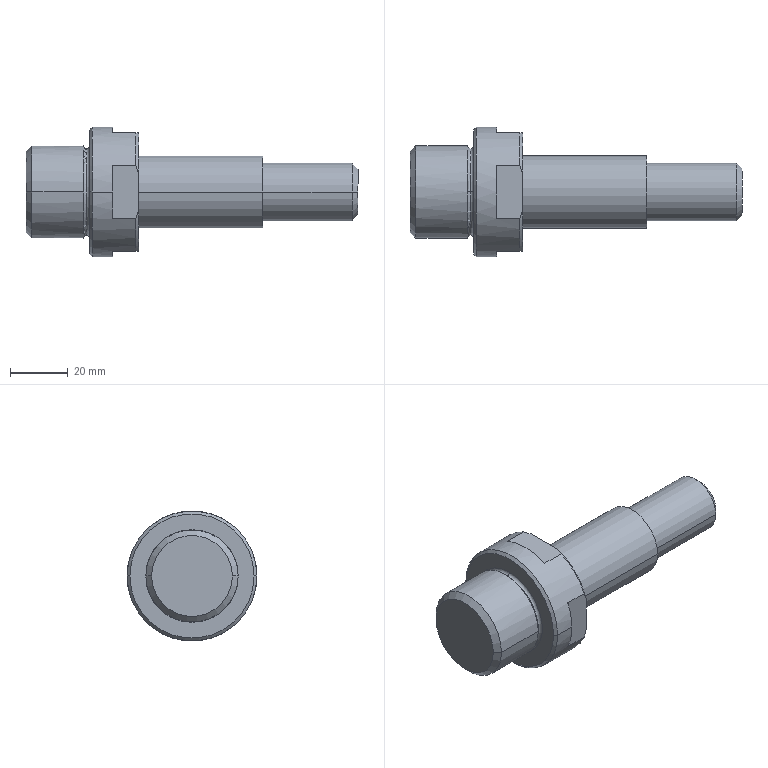Component | SolidWorks | FE5-226--a_b-1 | 1 solid | 35 faces | box 115 x 45 x 45 mm | volume 74739 mm3 | plane 13 | cone 10 | cylinder 8 | torus 4 | commonest cylinder face diameters 32 x2 20 x2 25 x2 45 x2
build123d program:
from build123d import *

# Parameters (mm, degrees)
SKETCH2_R       = 1
CHAMFER2_1_SIZE = 2
CHAMFER1_1_SIZE = 1
SKETCH3_W       = 30
SKETCH3_H       = 5
SKETCH3_W_2     = 5
SKETCH3_H_2     = 30
EXTRUDE1_DEPTH  = 9


with BuildPart() as part:
    # Sketch1 → Revolve1 (revolve)
    with BuildSketch(Plane(origin=(0, 0, 0), x_dir=(0, 0, -1), z_dir=(1, 0, 0))):
        Polygon((-115, 0), (-115, 16), (-93, 16), (-93, 22.5), (-76, 22.5), (-76, 12.5), (-33, 12.5), (-33, 10), (0, 10), (0, 0), align=None)
    revolve(axis=Axis((0, 0, 0), (0, 0, 1)))

    # Sketch2 → Cut-Revolve1 (revolve, cut)
    with BuildSketch(Plane(origin=(0, 0, 0), x_dir=(0, 0, -1), z_dir=(1, 0, 0)), mode=Mode.PRIVATE) as cut_revolve1_sk:
        with Locations((-94, 16)):
            Circle(SKETCH2_R)
    revolve(cut_revolve1_sk.sketch.rotate(Axis((0, 0, 0), (0, 0, 1)), 90), axis=Axis((0, 0, 0), (0, 0, 1)), mode=Mode.SUBTRACT)

    # Chamfer2-1
    chamfer2_1_edges = [part.edges().sort_by_distance(p)[0] for p in [
        (0, -16, 115),
        (0, -10, 0),
    ]]
    chamfer(chamfer2_1_edges, length=CHAMFER2_1_SIZE)

    # Chamfer1-1
    chamfer1_1_edges = [part.edges().sort_by_distance(p)[0] for p in [
        (0, -22.5, 76),
        (0, -22.5, 93),
    ]]
    chamfer(chamfer1_1_edges, length=CHAMFER1_1_SIZE)

    # Sketch3 → Extrude1 (cut)
    with BuildSketch(Plane(origin=(0, 0, 76), x_dir=(-1, 0, 0), z_dir=(0, 0, -1))):
        with Locations((0, 23)):
            Rectangle(SKETCH3_W, SKETCH3_H)
        with Locations((23, 0)):
            Rectangle(SKETCH3_W_2, SKETCH3_H_2)
        with Locations((-23, 0)):
            Rectangle(SKETCH3_W_2, SKETCH3_H_2)
        with Locations((0, -23)):
            Rectangle(SKETCH3_W, SKETCH3_H)
    extrude(amount=-EXTRUDE1_DEPTH, mode=Mode.SUBTRACT)


solid = part.part

# Placed as in the assembly
solid = solid.moved(Location((100, 81, -460), (0, -90, 0)))
STEP:
#1=CARTESIAN_POINT('',(0.2756,3.189,-18.74));
#2=VERTEX_POINT('',#1);
#3=CARTESIAN_POINT('',(0.2362,3.189,-18.701));
#4=VERTEX_POINT('',#3);
#5=CARTESIAN_POINT('',(0.2362,3.189,-18.74));
#6=DIRECTION('',(-0.,-1.,-0.));
#7=DIRECTION('',(1.,0.,0.));
#8=AXIS2_PLACEMENT_3D('',#5,#6,#7);
#9=CIRCLE('',#8,0.03937);
#10=EDGE_CURVE('',#2,#4,#9,.T.);
#11=ORIENTED_EDGE('',*,*,#10,.T.);
#12=CARTESIAN_POINT('',(0.2362,3.189,-17.52));
#13=VERTEX_POINT('',#12);
#14=CARTESIAN_POINT('',(0.2362,3.189,-18.11));
#15=DIRECTION('',(1.,-0.,-0.));
#16=DIRECTION('',(-0.,0.,-1.));
#17=AXIS2_PLACEMENT_3D('',#14,#15,#16);
#18=CIRCLE('',#17,0.5906);
#19=EDGE_CURVE('',#4,#13,#18,.T.);
#20=ORIENTED_EDGE('',*,*,#19,.T.);
#21=CARTESIAN_POINT('',(0.2756,3.189,-17.48));
#22=VERTEX_POINT('',#21);
#23=CARTESIAN_POINT('',(0.2362,3.189,-17.48));
#24=DIRECTION('',(0.,1.,-0.));
#25=DIRECTION('',(-1.,0.,0.));
#26=AXIS2_PLACEMENT_3D('',#23,#24,#25);
#27=CIRCLE('',#26,0.03937);
#28=EDGE_CURVE('',#22,#13,#27,.T.);
#29=ORIENTED_EDGE('',*,*,#28,.F.);
#30=CARTESIAN_POINT('',(0.2756,3.189,-18.11));
#31=DIRECTION('',(1.,-0.,-0.));
#32=DIRECTION('',(-0.,0.,-1.));
#33=AXIS2_PLACEMENT_3D('',#30,#31,#32);
#34=CIRCLE('',#33,0.6299);
#35=EDGE_CURVE('',#2,#22,#34,.T.);
#36=ORIENTED_EDGE('',*,*,#35,.F.);
#37=EDGE_LOOP('',(#11,#20,#29,#36));
#38=FACE_OUTER_BOUND('',#37,.T.);
#39=CARTESIAN_POINT('',(0.2362,3.189,-18.11));
#40=DIRECTION('',(1.,-0.,-0.));
#41=DIRECTION('',(-0.,0.,-1.));
#42=AXIS2_PLACEMENT_3D('',#39,#40,#41);
#43=TOROIDAL_SURFACE('',#42,0.6299,0.03937);
#44=ADVANCED_FACE('',(#38),#43,.F.);
#45=ORIENTED_EDGE('',*,*,#28,.T.);
#46=CARTESIAN_POINT('',(0.2362,3.189,-18.11));
#47=DIRECTION('',(1.,-0.,-0.));
#48=DIRECTION('',(-0.,0.,-1.));
#49=AXIS2_PLACEMENT_3D('',#46,#47,#48);
#50=CIRCLE('',#49,0.5906);
#51=EDGE_CURVE('',#13,#4,#50,.T.);
#52=ORIENTED_EDGE('',*,*,#51,.T.);
#53=ORIENTED_EDGE('',*,*,#10,.F.);
#54=CARTESIAN_POINT('',(0.2756,3.189,-18.11));
#55=DIRECTION('',(1.,-0.,-0.));
#56=DIRECTION('',(-0.,0.,-1.));
#57=AXIS2_PLACEMENT_3D('',#54,#55,#56);
#58=CIRCLE('',#57,0.6299);
#59=EDGE_CURVE('',#22,#2,#58,.T.);
#60=ORIENTED_EDGE('',*,*,#59,.F.);
#61=EDGE_LOOP('',(#45,#52,#53,#60));
#62=FACE_OUTER_BOUND('',#61,.T.);
#63=CARTESIAN_POINT('',(0.2362,3.189,-18.11));
#64=DIRECTION('',(1.,-0.,-0.));
#65=DIRECTION('',(-0.,0.,-1.));
#66=AXIS2_PLACEMENT_3D('',#63,#64,#65);
#67=TOROIDAL_SURFACE('',#66,0.6299,0.03937);
#68=ADVANCED_FACE('',(#62),#67,.F.);
#69=CARTESIAN_POINT('',(0.2756,2.343,-18.11));
#70=VERTEX_POINT('',#69);
#71=CARTESIAN_POINT('',(0.2756,4.035,-18.11));
#72=VERTEX_POINT('',#71);
#73=CARTESIAN_POINT('',(0.2756,3.189,-18.11));
#74=DIRECTION('',(-1.,0.,0.));
#75=DIRECTION('',(0.,-1.,0.));
#76=AXIS2_PLACEMENT_3D('',#73,#74,#75);
#77=CIRCLE('',#76,0.8465);
#78=EDGE_CURVE('',#70,#72,#77,.T.);
#79=ORIENTED_EDGE('',*,*,#78,.F.);
#80=CARTESIAN_POINT('',(0.315,2.303,-18.11));
#81=VERTEX_POINT('',#80);
#82=CARTESIAN_POINT('',(0.315,2.303,-18.11));
#83=DIRECTION('',(0.7071,-0.7071,-0.));
#84=VECTOR('',#83,39.37);
#85=LINE('',#82,#84);
#86=EDGE_CURVE('',#70,#81,#85,.T.);
#87=ORIENTED_EDGE('',*,*,#86,.T.);
#88=CARTESIAN_POINT('',(0.315,4.075,-18.11));
#89=VERTEX_POINT('',#88);
#90=CARTESIAN_POINT('',(0.315,3.189,-18.11));
#91=DIRECTION('',(1.,-0.,-0.));
#92=DIRECTION('',(0.,-1.,0.));
#93=AXIS2_PLACEMENT_3D('',#90,#91,#92);
#94=CIRCLE('',#93,0.8858);
#95=EDGE_CURVE('',#89,#81,#94,.T.);
#96=ORIENTED_EDGE('',*,*,#95,.F.);
#97=CARTESIAN_POINT('',(0.315,4.075,-18.11));
#98=DIRECTION('',(0.7071,0.7071,-0.));
#99=VECTOR('',#98,39.37);
#100=LINE('',#97,#99);
#101=EDGE_CURVE('',#72,#89,#100,.T.);
#102=ORIENTED_EDGE('',*,*,#101,.F.);
#103=EDGE_LOOP('',(#79,#87,#96,#102));
#104=FACE_OUTER_BOUND('',#103,.T.);
#105=CARTESIAN_POINT('',(0.315,3.189,-18.11));
#106=DIRECTION('',(1.,-0.,-0.));
#107=DIRECTION('',(0.,1.,0.));
#108=AXIS2_PLACEMENT_3D('',#105,#106,#107);
#109=CONICAL_SURFACE('',#108,0.8858,0.7854);
#110=ADVANCED_FACE('',(#104),#109,.T.);
#111=CARTESIAN_POINT('',(-0.5906,2.638,-18.11));
#112=VERTEX_POINT('',#111);
#113=CARTESIAN_POINT('',(-0.5906,3.74,-18.11));
#114=VERTEX_POINT('',#113);
#115=CARTESIAN_POINT('',(-0.5906,3.189,-18.11));
#116=DIRECTION('',(-1.,0.,0.));
#117=DIRECTION('',(0.,-1.,0.));
#118=AXIS2_PLACEMENT_3D('',#115,#116,#117);
#119=CIRCLE('',#118,0.5512);
#120=EDGE_CURVE('',#112,#114,#119,.T.);
#121=ORIENTED_EDGE('',*,*,#120,.F.);
#122=CARTESIAN_POINT('',(-0.5118,2.559,-18.11));
#123=VERTEX_POINT('',#122);
#124=CARTESIAN_POINT('',(-0.5118,2.559,-18.11));
#125=DIRECTION('',(0.7071,-0.7071,-0.));
#126=VECTOR('',#125,39.37);
#127=LINE('',#124,#126);
#128=EDGE_CURVE('',#112,#123,#127,.T.);
#129=ORIENTED_EDGE('',*,*,#128,.T.);
#130=CARTESIAN_POINT('',(-0.5118,3.819,-18.11));
#131=VERTEX_POINT('',#130);
#132=CARTESIAN_POINT('',(-0.5118,3.189,-18.11));
#133=DIRECTION('',(1.,0.,-0.));
#134=DIRECTION('',(0.,-1.,0.));
#135=AXIS2_PLACEMENT_3D('',#132,#133,#134);
#136=CIRCLE('',#135,0.6299);
#137=EDGE_CURVE('',#131,#123,#136,.T.);
#138=ORIENTED_EDGE('',*,*,#137,.F.);
#139=CARTESIAN_POINT('',(-0.5118,3.819,-18.11));
#140=DIRECTION('',(0.7071,0.7071,-0.));
#141=VECTOR('',#140,39.37);
#142=LINE('',#139,#141);
#143=EDGE_CURVE('',#114,#131,#142,.T.);
#144=ORIENTED_EDGE('',*,*,#143,.F.);
#145=EDGE_LOOP('',(#121,#129,#138,#144));
#146=FACE_OUTER_BOUND('',#145,.T.);
#147=CARTESIAN_POINT('',(-0.5118,3.189,-18.11));
#148=DIRECTION('',(1.,0.,-0.));
#149=DIRECTION('',(0.,1.,0.));
#150=AXIS2_PLACEMENT_3D('',#147,#148,#149);
#151=CONICAL_SURFACE('',#150,0.6299,0.7854);
#152=ADVANCED_FACE('',(#146),#151,.T.);
#153=CARTESIAN_POINT('',(3.937,3.504,-18.11));
#154=VERTEX_POINT('',#153);
#155=CARTESIAN_POINT('',(3.937,2.874,-18.11));
#156=VERTEX_POINT('',#155);
#157=CARTESIAN_POINT('',(3.937,3.189,-18.11));
#158=DIRECTION('',(1.,-0.,-0.));
#159=DIRECTION('',(0.,1.,0.));
#160=AXIS2_PLACEMENT_3D('',#157,#158,#159);
#161=CIRCLE('',#160,0.315);
#162=EDGE_CURVE('',#154,#156,#161,.T.);
#163=ORIENTED_EDGE('',*,*,#162,.F.);
#164=CARTESIAN_POINT('',(3.858,3.583,-18.11));
#165=VERTEX_POINT('',#164);
#166=CARTESIAN_POINT('',(3.937,3.504,-18.11));
#167=DIRECTION('',(-0.7071,0.7071,0.));
#168=VECTOR('',#167,39.37);
#169=LINE('',#166,#168);
#170=EDGE_CURVE('',#154,#165,#169,.T.);
#171=ORIENTED_EDGE('',*,*,#170,.T.);
#172=CARTESIAN_POINT('',(3.858,2.795,-18.11));
#173=VERTEX_POINT('',#172);
#174=CARTESIAN_POINT('',(3.858,3.189,-18.11));
#175=DIRECTION('',(-1.,0.,0.));
#176=DIRECTION('',(0.,1.,0.));
#177=AXIS2_PLACEMENT_3D('',#174,#175,#176);
#178=CIRCLE('',#177,0.3937);
#179=EDGE_CURVE('',#173,#165,#178,.T.);
#180=ORIENTED_EDGE('',*,*,#179,.F.);
#181=CARTESIAN_POINT('',(3.937,2.874,-18.11));
#182=DIRECTION('',(-0.7071,-0.7071,0.));
#183=VECTOR('',#182,39.37);
#184=LINE('',#181,#183);
#185=EDGE_CURVE('',#156,#173,#184,.T.);
#186=ORIENTED_EDGE('',*,*,#185,.F.);
#187=EDGE_LOOP('',(#163,#171,#180,#186));
#188=FACE_OUTER_BOUND('',#187,.T.);
#189=CARTESIAN_POINT('',(3.937,3.189,-18.11));
#190=DIRECTION('',(-1.,0.,0.));
#191=DIRECTION('',(0.,-1.,0.));
#192=AXIS2_PLACEMENT_3D('',#189,#190,#191);
#193=CONICAL_SURFACE('',#192,0.315,0.7854);
#194=ADVANCED_FACE('',(#188),#193,.T.);
#195=ORIENTED_EDGE('',*,*,#137,.T.);
#196=CARTESIAN_POINT('',(0.1969,2.559,-18.11));
#197=VERTEX_POINT('',#196);
#198=CARTESIAN_POINT('',(3.937,2.559,-18.11));
#199=DIRECTION('',(1.,-0.,-0.));
#200=VECTOR('',#199,39.37);
#201=LINE('',#198,#200);
#202=EDGE_CURVE('',#123,#197,#201,.T.);
#203=ORIENTED_EDGE('',*,*,#202,.T.);
#204=CARTESIAN_POINT('',(0.1969,3.189,-17.48));
#205=VERTEX_POINT('',#204);
#206=CARTESIAN_POINT('',(0.1969,3.189,-18.11));
#207=DIRECTION('',(1.,-0.,-0.));
#208=DIRECTION('',(-0.,0.,-1.));
#209=AXIS2_PLACEMENT_3D('',#206,#207,#208);
#210=CIRCLE('',#209,0.6299);
#211=EDGE_CURVE('',#205,#197,#210,.T.);
#212=ORIENTED_EDGE('',*,*,#211,.F.);
#213=CARTESIAN_POINT('',(0.1969,3.819,-18.11));
#214=VERTEX_POINT('',#213);
#215=CARTESIAN_POINT('',(0.1969,3.189,-18.11));
#216=DIRECTION('',(1.,-0.,-0.));
#217=DIRECTION('',(-0.,0.,-1.));
#218=AXIS2_PLACEMENT_3D('',#215,#216,#217);
#219=CIRCLE('',#218,0.6299);
#220=EDGE_CURVE('',#214,#205,#219,.T.);
#221=ORIENTED_EDGE('',*,*,#220,.F.);
#222=CARTESIAN_POINT('',(3.937,3.819,-18.11));
#223=DIRECTION('',(1.,-0.,-0.));
#224=VECTOR('',#223,39.37);
#225=LINE('',#222,#224);
#226=EDGE_CURVE('',#131,#214,#225,.T.);
#227=ORIENTED_EDGE('',*,*,#226,.F.);
#228=EDGE_LOOP('',(#195,#203,#212,#221,#227));
#229=FACE_OUTER_BOUND('',#228,.T.);
#230=CARTESIAN_POINT('',(3.937,3.189,-18.11));
#231=DIRECTION('',(1.,-0.,-0.));
#232=DIRECTION('',(0.,1.,0.));
#233=AXIS2_PLACEMENT_3D('',#230,#231,#232);
#234=CYLINDRICAL_SURFACE('',#233,0.6299);
#235=ADVANCED_FACE('',(#229),#234,.T.);
#236=ORIENTED_EDGE('',*,*,#51,.F.);
#237=CARTESIAN_POINT('',(0.2362,3.189,-17.48));
#238=DIRECTION('',(0.,1.,-0.));
#239=DIRECTION('',(-1.,0.,0.));
#240=AXIS2_PLACEMENT_3D('',#237,#238,#239);
#241=CIRCLE('',#240,0.03937);
#242=EDGE_CURVE('',#13,#205,#241,.T.);
#243=ORIENTED_EDGE('',*,*,#242,.T.);
#244=ORIENTED_EDGE('',*,*,#211,.T.);
#245=CARTESIAN_POINT('',(0.1969,3.189,-18.74));
#246=VERTEX_POINT('',#245);
#247=CARTESIAN_POINT('',(0.1969,3.189,-18.11));
#248=DIRECTION('',(1.,-0.,-0.));
#249=DIRECTION('',(-0.,0.,-1.));
#250=AXIS2_PLACEMENT_3D('',#247,#248,#249);
#251=CIRCLE('',#250,0.6299);
#252=EDGE_CURVE('',#197,#246,#251,.T.);
#253=ORIENTED_EDGE('',*,*,#252,.T.);
#254=CARTESIAN_POINT('',(0.2362,3.189,-18.74));
#255=DIRECTION('',(-0.,-1.,-0.));
#256=DIRECTION('',(1.,0.,0.));
#257=AXIS2_PLACEMENT_3D('',#254,#255,#256);
#258=CIRCLE('',#257,0.03937);
#259=EDGE_CURVE('',#4,#246,#258,.T.);
#260=ORIENTED_EDGE('',*,*,#259,.F.);
#261=EDGE_LOOP('',(#236,#243,#244,#253,#260));
#262=FACE_OUTER_BOUND('',#261,.T.);
#263=CARTESIAN_POINT('',(0.2362,3.189,-18.11));
#264=DIRECTION('',(1.,-0.,-0.));
#265=DIRECTION('',(-0.,0.,-1.));
#266=AXIS2_PLACEMENT_3D('',#263,#264,#265);
#267=TOROIDAL_SURFACE('',#266,0.6299,0.03937);
#268=ADVANCED_FACE('',(#262),#267,.F.);
#269=CARTESIAN_POINT('',(2.638,3.583,-18.11));
#270=VERTEX_POINT('',#269);
#271=CARTESIAN_POINT('',(2.638,2.795,-18.11));
#272=VERTEX_POINT('',#271);
#273=CARTESIAN_POINT('',(2.638,3.189,-18.11));
#274=DIRECTION('',(1.,-0.,-0.));
#275=DIRECTION('',(0.,1.,0.));
#276=AXIS2_PLACEMENT_3D('',#273,#274,#275);
#277=CIRCLE('',#276,0.3937);
#278=EDGE_CURVE('',#270,#272,#277,.T.);
#279=ORIENTED_EDGE('',*,*,#278,.T.);
#280=CARTESIAN_POINT('',(3.937,2.795,-18.11));
#281=DIRECTION('',(1.,-0.,-0.));
#282=VECTOR('',#281,39.37);
#283=LINE('',#280,#282);
#284=EDGE_CURVE('',#272,#173,#283,.T.);
#285=ORIENTED_EDGE('',*,*,#284,.T.);
#286=ORIENTED_EDGE('',*,*,#179,.T.);
#287=CARTESIAN_POINT('',(3.937,3.583,-18.11));
#288=DIRECTION('',(1.,-0.,-0.));
#289=VECTOR('',#288,39.37);
#290=LINE('',#287,#289);
#291=EDGE_CURVE('',#270,#165,#290,.T.);
#292=ORIENTED_EDGE('',*,*,#291,.F.);
#293=EDGE_LOOP('',(#279,#285,#286,#292));
#294=FACE_OUTER_BOUND('',#293,.T.);
#295=CARTESIAN_POINT('',(3.937,3.189,-18.11));
#296=DIRECTION('',(1.,-0.,-0.));
#297=DIRECTION('',(0.,1.,0.));
#298=AXIS2_PLACEMENT_3D('',#295,#296,#297);
#299=CYLINDRICAL_SURFACE('',#298,0.3937);
#300=ADVANCED_FACE('',(#294),#299,.T.);
#301=CARTESIAN_POINT('',(0.9449,3.681,-18.11));
#302=VERTEX_POINT('',#301);
#303=CARTESIAN_POINT('',(0.9449,2.697,-18.11));
#304=VERTEX_POINT('',#303);
#305=CARTESIAN_POINT('',(0.9449,3.189,-18.11));
#306=DIRECTION('',(1.,-0.,-0.));
#307=DIRECTION('',(0.,1.,0.));
#308=AXIS2_PLACEMENT_3D('',#305,#306,#307);
#309=CIRCLE('',#308,0.4921);
#310=EDGE_CURVE('',#302,#304,#309,.T.);
#311=ORIENTED_EDGE('',*,*,#310,.T.);
#312=CARTESIAN_POINT('',(2.638,2.697,-18.11));
#313=VERTEX_POINT('',#312);
#314=CARTESIAN_POINT('',(3.937,2.697,-18.11));
#315=DIRECTION('',(1.,-0.,-0.));
#316=VECTOR('',#315,39.37);
#317=LINE('',#314,#316);
#318=EDGE_CURVE('',#304,#313,#317,.T.);
#319=ORIENTED_EDGE('',*,*,#318,.T.);
#320=CARTESIAN_POINT('',(2.638,3.681,-18.11));
#321=VERTEX_POINT('',#320);
#322=CARTESIAN_POINT('',(2.638,3.189,-18.11));
#323=DIRECTION('',(1.,-0.,-0.));
#324=DIRECTION('',(0.,1.,0.));
#325=AXIS2_PLACEMENT_3D('',#322,#323,#324);
#326=CIRCLE('',#325,0.4921);
#327=EDGE_CURVE('',#321,#313,#326,.T.);
#328=ORIENTED_EDGE('',*,*,#327,.F.);
#329=CARTESIAN_POINT('',(3.937,3.681,-18.11));
#330=DIRECTION('',(1.,-0.,-0.));
#331=VECTOR('',#330,39.37);
#332=LINE('',#329,#331);
#333=EDGE_CURVE('',#302,#321,#332,.T.);
#334=ORIENTED_EDGE('',*,*,#333,.F.);
#335=EDGE_LOOP('',(#311,#319,#328,#334));
#336=FACE_OUTER_BOUND('',#335,.T.);
#337=CARTESIAN_POINT('',(3.937,3.189,-18.11));
#338=DIRECTION('',(1.,-0.,-0.));
#339=DIRECTION('',(0.,1.,0.));
#340=AXIS2_PLACEMENT_3D('',#337,#338,#339);
#341=CYLINDRICAL_SURFACE('',#340,0.4921);
#342=ADVANCED_FACE('',(#336),#341,.T.);
#343=ORIENTED_EDGE('',*,*,#95,.T.);
#344=CARTESIAN_POINT('',(0.5906,2.303,-18.11));
#345=VERTEX_POINT('',#344);
#346=CARTESIAN_POINT('',(3.937,2.303,-18.11));
#347=DIRECTION('',(1.,-0.,-0.));
#348=VECTOR('',#347,39.37);
#349=LINE('',#346,#348);
#350=EDGE_CURVE('',#81,#345,#349,.T.);
#351=ORIENTED_EDGE('',*,*,#350,.T.);
#352=CARTESIAN_POINT('',(0.5906,2.382,-17.745));
#353=VERTEX_POINT('',#352);
#354=CARTESIAN_POINT('',(0.5906,3.189,-18.11));
#355=DIRECTION('',(-1.,0.,0.));
#356=DIRECTION('',(-0.,0.,-1.));
#357=AXIS2_PLACEMENT_3D('',#354,#355,#356);
#358=CIRCLE('',#357,0.8858);
#359=EDGE_CURVE('',#345,#353,#358,.T.);
#360=ORIENTED_EDGE('',*,*,#359,.T.);
#361=CARTESIAN_POINT('',(0.9055,2.382,-17.745));
#362=VERTEX_POINT('',#361);
#363=CARTESIAN_POINT('',(3.937,2.382,-17.745));
#364=DIRECTION('',(-1.,0.,0.));
#365=VECTOR('',#364,39.37);
#366=LINE('',#363,#365);
#367=EDGE_CURVE('',#362,#353,#366,.T.);
#368=ORIENTED_EDGE('',*,*,#367,.F.);
#369=CARTESIAN_POINT('',(0.9055,2.824,-17.303));
#370=VERTEX_POINT('',#369);
#371=CARTESIAN_POINT('',(0.9055,3.189,-18.11));
#372=DIRECTION('',(-1.,0.,0.));
#373=DIRECTION('',(0.,1.,-0.));
#374=AXIS2_PLACEMENT_3D('',#371,#372,#373);
#375=CIRCLE('',#374,0.8858);
#376=EDGE_CURVE('',#362,#370,#375,.T.);
#377=ORIENTED_EDGE('',*,*,#376,.T.);
#378=CARTESIAN_POINT('',(0.5906,2.824,-17.303));
#379=VERTEX_POINT('',#378);
#380=CARTESIAN_POINT('',(3.937,2.824,-17.303));
#381=DIRECTION('',(1.,-0.,-0.));
#382=VECTOR('',#381,39.37);
#383=LINE('',#380,#382);
#384=EDGE_CURVE('',#379,#370,#383,.T.);
#385=ORIENTED_EDGE('',*,*,#384,.F.);
#386=CARTESIAN_POINT('',(0.5906,3.554,-17.303));
#387=VERTEX_POINT('',#386);
#388=CARTESIAN_POINT('',(0.5906,3.189,-18.11));
#389=DIRECTION('',(-1.,0.,0.));
#390=DIRECTION('',(-0.,0.,-1.));
#391=AXIS2_PLACEMENT_3D('',#388,#389,#390);
#392=CIRCLE('',#391,0.8858);
#393=EDGE_CURVE('',#379,#387,#392,.T.);
#394=ORIENTED_EDGE('',*,*,#393,.T.);
#395=CARTESIAN_POINT('',(0.9055,3.554,-17.303));
#396=VERTEX_POINT('',#395);
#397=CARTESIAN_POINT('',(3.937,3.554,-17.303));
#398=DIRECTION('',(-1.,0.,0.));
#399=VECTOR('',#398,39.37);
#400=LINE('',#397,#399);
#401=EDGE_CURVE('',#396,#387,#400,.T.);
#402=ORIENTED_EDGE('',*,*,#401,.F.);
#403=CARTESIAN_POINT('',(0.9055,3.996,-17.745));
#404=VERTEX_POINT('',#403);
#405=CARTESIAN_POINT('',(0.9055,3.189,-18.11));
#406=DIRECTION('',(-1.,0.,0.));
#407=DIRECTION('',(0.,1.,-0.));
#408=AXIS2_PLACEMENT_3D('',#405,#406,#407);
#409=CIRCLE('',#408,0.8858);
#410=EDGE_CURVE('',#396,#404,#409,.T.);
#411=ORIENTED_EDGE('',*,*,#410,.T.);
#412=CARTESIAN_POINT('',(0.5906,3.996,-17.745));
#413=VERTEX_POINT('',#412);
#414=CARTESIAN_POINT('',(3.937,3.996,-17.745));
#415=DIRECTION('',(1.,-0.,-0.));
#416=VECTOR('',#415,39.37);
#417=LINE('',#414,#416);
#418=EDGE_CURVE('',#413,#404,#417,.T.);
#419=ORIENTED_EDGE('',*,*,#418,.F.);
#420=CARTESIAN_POINT('',(0.5906,4.075,-18.11));
#421=VERTEX_POINT('',#420);
#422=CARTESIAN_POINT('',(0.5906,3.189,-18.11));
#423=DIRECTION('',(-1.,0.,0.));
#424=DIRECTION('',(-0.,-0.,-1.));
#425=AXIS2_PLACEMENT_3D('',#422,#423,#424);
#426=CIRCLE('',#425,0.8858);
#427=EDGE_CURVE('',#413,#421,#426,.T.);
#428=ORIENTED_EDGE('',*,*,#427,.T.);
#429=CARTESIAN_POINT('',(3.937,4.075,-18.11));
#430=DIRECTION('',(1.,-0.,-0.));
#431=VECTOR('',#430,39.37);
#432=LINE('',#429,#431);
#433=EDGE_CURVE('',#89,#421,#432,.T.);
#434=ORIENTED_EDGE('',*,*,#433,.F.);
#435=EDGE_LOOP('',(#343,#351,#360,#368,#377,#385,#394,#402,#411,#419,#428,#434));
#436=FACE_OUTER_BOUND('',#435,.T.);
#437=CARTESIAN_POINT('',(3.937,3.189,-18.11));
#438=DIRECTION('',(1.,-0.,-0.));
#439=DIRECTION('',(0.,1.,0.));
#440=AXIS2_PLACEMENT_3D('',#437,#438,#439);
#441=CYLINDRICAL_SURFACE('',#440,0.8858);
#442=ADVANCED_FACE('',(#436),#441,.T.);
#443=CARTESIAN_POINT('',(0.9055,2.382,-18.475));
#444=VERTEX_POINT('',#443);
#445=CARTESIAN_POINT('',(0.9449,2.382,-18.365));
#446=VERTEX_POINT('',#445);
#447=CARTESIAN_POINT('',(0.9055,2.382,-18.475));
#448=CARTESIAN_POINT('',(0.9203,2.382,-18.44));
#449=CARTESIAN_POINT('',(0.9335,2.382,-18.403));
#450=CARTESIAN_POINT('',(0.9449,2.382,-18.365));
#451=B_SPLINE_CURVE_WITH_KNOTS('',3,(#447,#448,#449,#450),.UNSPECIFIED.,.F.,.F.,(4,4),(0.02898,0.03193),.UNSPECIFIED.);
#452=EDGE_CURVE('',#444,#446,#451,.T.);
#453=ORIENTED_EDGE('',*,*,#452,.F.);
#454=CARTESIAN_POINT('',(0.9055,2.824,-18.917));
#455=VERTEX_POINT('',#454);
#456=CARTESIAN_POINT('',(0.9055,3.189,-18.11));
#457=DIRECTION('',(-1.,0.,0.));
#458=DIRECTION('',(0.,1.,0.));
#459=AXIS2_PLACEMENT_3D('',#456,#457,#458);
#460=CIRCLE('',#459,0.8858);
#461=EDGE_CURVE('',#455,#444,#460,.T.);
#462=ORIENTED_EDGE('',*,*,#461,.F.);
#463=CARTESIAN_POINT('',(0.9449,2.934,-18.917));
#464=VERTEX_POINT('',#463);
#465=CARTESIAN_POINT('',(0.9449,2.934,-18.917));
#466=CARTESIAN_POINT('',(0.9337,2.897,-18.917));
#467=CARTESIAN_POINT('',(0.9204,2.86,-18.917));
#468=CARTESIAN_POINT('',(0.9055,2.824,-18.917));
#469=B_SPLINE_CURVE_WITH_KNOTS('',3,(#465,#466,#467,#468),.UNSPECIFIED.,.F.,.F.,(4,4),(0.04504,0.04799),.UNSPECIFIED.);
#470=EDGE_CURVE('',#464,#455,#469,.T.);
#471=ORIENTED_EDGE('',*,*,#470,.F.);
#472=CARTESIAN_POINT('',(0.9449,3.189,-18.11));
#473=DIRECTION('',(1.,-0.,-0.));
#474=DIRECTION('',(0.,1.,0.));
#475=AXIS2_PLACEMENT_3D('',#472,#473,#474);
#476=CIRCLE('',#475,0.8465);
#477=EDGE_CURVE('',#446,#464,#476,.T.);
#478=ORIENTED_EDGE('',*,*,#477,.F.);
#479=EDGE_LOOP('',(#453,#462,#471,#478));
#480=FACE_OUTER_BOUND('',#479,.T.);
#481=CARTESIAN_POINT('',(0.9449,3.189,-18.11));
#482=DIRECTION('',(-1.,0.,0.));
#483=DIRECTION('',(0.,-1.,0.));
#484=AXIS2_PLACEMENT_3D('',#481,#482,#483);
#485=CONICAL_SURFACE('',#484,0.8465,0.7854);
#486=ADVANCED_FACE('',(#480),#485,.T.);
#487=CARTESIAN_POINT('',(0.9449,2.382,-17.855));
#488=VERTEX_POINT('',#487);
#489=CARTESIAN_POINT('',(0.9449,2.382,-17.855));
#490=CARTESIAN_POINT('',(0.9337,2.382,-17.818));
#491=CARTESIAN_POINT('',(0.9204,2.382,-17.781));
#492=CARTESIAN_POINT('',(0.9055,2.382,-17.745));
#493=B_SPLINE_CURVE_WITH_KNOTS('',3,(#489,#490,#491,#492),.UNSPECIFIED.,.F.,.F.,(4,4),(0.04504,0.04799),.UNSPECIFIED.);
#494=EDGE_CURVE('',#488,#362,#493,.T.);
#495=ORIENTED_EDGE('',*,*,#494,.F.);
#496=CARTESIAN_POINT('',(0.9449,2.934,-17.303));
#497=VERTEX_POINT('',#496);
#498=CARTESIAN_POINT('',(0.9449,3.189,-18.11));
#499=DIRECTION('',(1.,-0.,-0.));
#500=DIRECTION('',(0.,1.,0.));
#501=AXIS2_PLACEMENT_3D('',#498,#499,#500);
#502=CIRCLE('',#501,0.8465);
#503=EDGE_CURVE('',#497,#488,#502,.T.);
#504=ORIENTED_EDGE('',*,*,#503,.F.);
#505=CARTESIAN_POINT('',(0.9055,2.824,-17.303));
#506=CARTESIAN_POINT('',(0.9203,2.86,-17.303));
#507=CARTESIAN_POINT('',(0.9335,2.896,-17.303));
#508=CARTESIAN_POINT('',(0.9449,2.934,-17.303));
#509=B_SPLINE_CURVE_WITH_KNOTS('',3,(#505,#506,#507,#508),.UNSPECIFIED.,.F.,.F.,(4,4),(0.02898,0.03193),.UNSPECIFIED.);
#510=EDGE_CURVE('',#370,#497,#509,.T.);
#511=ORIENTED_EDGE('',*,*,#510,.F.);
#512=ORIENTED_EDGE('',*,*,#376,.F.);
#513=EDGE_LOOP('',(#495,#504,#511,#512));
#514=FACE_OUTER_BOUND('',#513,.T.);
#515=CARTESIAN_POINT('',(0.9449,3.189,-18.11));
#516=DIRECTION('',(-1.,0.,0.));
#517=DIRECTION('',(0.,-1.,0.));
#518=AXIS2_PLACEMENT_3D('',#515,#516,#517);
#519=CONICAL_SURFACE('',#518,0.8465,0.7854);
#520=ADVANCED_FACE('',(#514),#519,.T.);
#521=CARTESIAN_POINT('',(0.9055,3.554,-18.917));
#522=VERTEX_POINT('',#521);
#523=CARTESIAN_POINT('',(0.9449,3.444,-18.917));
#524=VERTEX_POINT('',#523);
#525=CARTESIAN_POINT('',(0.9055,3.554,-18.917));
#526=CARTESIAN_POINT('',(0.9203,3.518,-18.917));
#527=CARTESIAN_POINT('',(0.9335,3.482,-18.917));
#528=CARTESIAN_POINT('',(0.9449,3.444,-18.917));
#529=B_SPLINE_CURVE_WITH_KNOTS('',3,(#525,#526,#527,#528),.UNSPECIFIED.,.F.,.F.,(4,4),(0.02898,0.03193),.UNSPECIFIED.);
#530=EDGE_CURVE('',#522,#524,#529,.T.);
#531=ORIENTED_EDGE('',*,*,#530,.F.);
#532=CARTESIAN_POINT('',(0.9055,3.996,-18.475));
#533=VERTEX_POINT('',#532);
#534=CARTESIAN_POINT('',(0.9055,3.189,-18.11));
#535=DIRECTION('',(-1.,0.,0.));
#536=DIRECTION('',(0.,1.,0.));
#537=AXIS2_PLACEMENT_3D('',#534,#535,#536);
#538=CIRCLE('',#537,0.8858);
#539=EDGE_CURVE('',#533,#522,#538,.T.);
#540=ORIENTED_EDGE('',*,*,#539,.F.);
#541=CARTESIAN_POINT('',(0.9449,3.996,-18.365));
#542=VERTEX_POINT('',#541);
#543=CARTESIAN_POINT('',(0.9449,3.996,-18.365));
#544=CARTESIAN_POINT('',(0.9337,3.996,-18.403));
#545=CARTESIAN_POINT('',(0.9204,3.996,-18.439));
#546=CARTESIAN_POINT('',(0.9055,3.996,-18.475));
#547=B_SPLINE_CURVE_WITH_KNOTS('',3,(#543,#544,#545,#546),.UNSPECIFIED.,.F.,.F.,(4,4),(0.04504,0.04799),.UNSPECIFIED.);
#548=EDGE_CURVE('',#542,#533,#547,.T.);
#549=ORIENTED_EDGE('',*,*,#548,.F.);
#550=CARTESIAN_POINT('',(0.9449,3.189,-18.11));
#551=DIRECTION('',(1.,-0.,-0.));
#552=DIRECTION('',(0.,1.,0.));
#553=AXIS2_PLACEMENT_3D('',#550,#551,#552);
#554=CIRCLE('',#553,0.8465);
#555=EDGE_CURVE('',#524,#542,#554,.T.);
#556=ORIENTED_EDGE('',*,*,#555,.F.);
#557=EDGE_LOOP('',(#531,#540,#549,#556));
#558=FACE_OUTER_BOUND('',#557,.T.);
#559=CARTESIAN_POINT('',(0.9449,3.189,-18.11));
#560=DIRECTION('',(-1.,0.,0.));
#561=DIRECTION('',(0.,-1.,0.));
#562=AXIS2_PLACEMENT_3D('',#559,#560,#561);
#563=CONICAL_SURFACE('',#562,0.8465,0.7854);
#564=ADVANCED_FACE('',(#558),#563,.T.);
#565=CARTESIAN_POINT('',(0.2756,3.189,-18.11));
#566=DIRECTION('',(-1.,0.,0.));
#567=DIRECTION('',(0.,-1.,0.));
#568=AXIS2_PLACEMENT_3D('',#565,#566,#567);
#569=CIRCLE('',#568,0.8465);
#570=EDGE_CURVE('',#72,#70,#569,.T.);
#571=ORIENTED_EDGE('',*,*,#570,.T.);
#572=ORIENTED_EDGE('',*,*,#78,.T.);
#573=EDGE_LOOP('',(#571,#572));
#574=FACE_OUTER_BOUND('',#573,.T.);
#575=ORIENTED_EDGE('',*,*,#35,.T.);
#576=ORIENTED_EDGE('',*,*,#59,.T.);
#577=EDGE_LOOP('',(#575,#576));
#578=FACE_BOUND('',#577,.T.);
#579=CARTESIAN_POINT('',(0.2756,3.819,-18.11));
#580=DIRECTION('',(-1.,-0.,0.));
#581=DIRECTION('',(-0.,-1.,-0.));
#582=AXIS2_PLACEMENT_3D('',#579,#580,#581);
#583=PLANE('',#582);
#584=ADVANCED_FACE('',(#574,#578),#583,.T.);
#585=ORIENTED_EDGE('',*,*,#350,.F.);
#586=CARTESIAN_POINT('',(0.315,3.189,-18.11));
#587=DIRECTION('',(1.,-0.,-0.));
#588=DIRECTION('',(0.,-1.,-0.));
#589=AXIS2_PLACEMENT_3D('',#586,#587,#588);
#590=CIRCLE('',#589,0.8858);
#591=EDGE_CURVE('',#81,#89,#590,.T.);
#592=ORIENTED_EDGE('',*,*,#591,.T.);
#593=ORIENTED_EDGE('',*,*,#433,.T.);
#594=CARTESIAN_POINT('',(0.5906,3.996,-18.475));
#595=VERTEX_POINT('',#594);
#596=CARTESIAN_POINT('',(0.5906,3.189,-18.11));
#597=DIRECTION('',(-1.,0.,0.));
#598=DIRECTION('',(-0.,-0.,-1.));
#599=AXIS2_PLACEMENT_3D('',#596,#597,#598);
#600=CIRCLE('',#599,0.8858);
#601=EDGE_CURVE('',#421,#595,#600,.T.);
#602=ORIENTED_EDGE('',*,*,#601,.T.);
#603=CARTESIAN_POINT('',(3.937,3.996,-18.475));
#604=DIRECTION('',(-1.,0.,0.));
#605=VECTOR('',#604,39.37);
#606=LINE('',#603,#605);
#607=EDGE_CURVE('',#533,#595,#606,.T.);
#608=ORIENTED_EDGE('',*,*,#607,.F.);
#609=ORIENTED_EDGE('',*,*,#539,.T.);
#610=CARTESIAN_POINT('',(0.5906,3.554,-18.917));
#611=VERTEX_POINT('',#610);
#612=CARTESIAN_POINT('',(3.937,3.554,-18.917));
#613=DIRECTION('',(1.,-0.,-0.));
#614=VECTOR('',#613,39.37);
#615=LINE('',#612,#614);
#616=EDGE_CURVE('',#611,#522,#615,.T.);
#617=ORIENTED_EDGE('',*,*,#616,.F.);
#618=CARTESIAN_POINT('',(0.5906,2.824,-18.917));
#619=VERTEX_POINT('',#618);
#620=CARTESIAN_POINT('',(0.5906,3.189,-18.11));
#621=DIRECTION('',(-1.,0.,0.));
#622=DIRECTION('',(-0.,0.,-1.));
#623=AXIS2_PLACEMENT_3D('',#620,#621,#622);
#624=CIRCLE('',#623,0.8858);
#625=EDGE_CURVE('',#611,#619,#624,.T.);
#626=ORIENTED_EDGE('',*,*,#625,.T.);
#627=CARTESIAN_POINT('',(3.937,2.824,-18.917));
#628=DIRECTION('',(-1.,0.,0.));
#629=VECTOR('',#628,39.37);
#630=LINE('',#627,#629);
#631=EDGE_CURVE('',#455,#619,#630,.T.);
#632=ORIENTED_EDGE('',*,*,#631,.F.);
#633=ORIENTED_EDGE('',*,*,#461,.T.);
#634=CARTESIAN_POINT('',(0.5906,2.382,-18.475));
#635=VERTEX_POINT('',#634);
#636=CARTESIAN_POINT('',(3.937,2.382,-18.475));
#637=DIRECTION('',(1.,-0.,-0.));
#638=VECTOR('',#637,39.37);
#639=LINE('',#636,#638);
#640=EDGE_CURVE('',#635,#444,#639,.T.);
#641=ORIENTED_EDGE('',*,*,#640,.F.);
#642=CARTESIAN_POINT('',(0.5906,3.189,-18.11));
#643=DIRECTION('',(-1.,0.,0.));
#644=DIRECTION('',(-0.,-0.,-1.));
#645=AXIS2_PLACEMENT_3D('',#642,#643,#644);
#646=CIRCLE('',#645,0.8858);
#647=EDGE_CURVE('',#635,#345,#646,.T.);
#648=ORIENTED_EDGE('',*,*,#647,.T.);
#649=EDGE_LOOP('',(#585,#592,#593,#602,#608,#609,#617,#626,#632,#633,#641,#648));
#650=FACE_OUTER_BOUND('',#649,.T.);
#651=CARTESIAN_POINT('',(3.937,3.189,-18.11));
#652=DIRECTION('',(1.,-0.,-0.));
#653=DIRECTION('',(0.,1.,0.));
#654=AXIS2_PLACEMENT_3D('',#651,#652,#653);
#655=CYLINDRICAL_SURFACE('',#654,0.8858);
#656=ADVANCED_FACE('',(#650),#655,.T.);
#657=CARTESIAN_POINT('',(0.9449,2.382,-18.11));
#658=DIRECTION('',(0.,0.,1.));
#659=VECTOR('',#658,39.37);
#660=LINE('',#657,#659);
#661=EDGE_CURVE('',#446,#488,#660,.T.);
#662=ORIENTED_EDGE('',*,*,#661,.F.);
#663=ORIENTED_EDGE('',*,*,#477,.T.);
#664=CARTESIAN_POINT('',(0.9449,3.78,-18.917));
#665=DIRECTION('',(-0.,-1.,-0.));
#666=VECTOR('',#665,39.37);
#667=LINE('',#664,#666);
#668=EDGE_CURVE('',#524,#464,#667,.T.);
#669=ORIENTED_EDGE('',*,*,#668,.F.);
#670=ORIENTED_EDGE('',*,*,#555,.T.);
#671=CARTESIAN_POINT('',(0.9449,3.996,-17.855));
#672=VERTEX_POINT('',#671);
#673=CARTESIAN_POINT('',(0.9449,3.996,-17.52));
#674=DIRECTION('',(-0.,0.,-1.));
#675=VECTOR('',#674,39.37);
#676=LINE('',#673,#675);
#677=EDGE_CURVE('',#672,#542,#676,.T.);
#678=ORIENTED_EDGE('',*,*,#677,.F.);
#679=CARTESIAN_POINT('',(0.9449,3.444,-17.303));
#680=VERTEX_POINT('',#679);
#681=CARTESIAN_POINT('',(0.9449,3.189,-18.11));
#682=DIRECTION('',(1.,-0.,-0.));
#683=DIRECTION('',(0.,1.,0.));
#684=AXIS2_PLACEMENT_3D('',#681,#682,#683);
#685=CIRCLE('',#684,0.8465);
#686=EDGE_CURVE('',#672,#680,#685,.T.);
#687=ORIENTED_EDGE('',*,*,#686,.T.);
#688=CARTESIAN_POINT('',(0.9449,3.78,-17.303));
#689=DIRECTION('',(0.,1.,0.));
#690=VECTOR('',#689,39.37);
#691=LINE('',#688,#690);
#692=EDGE_CURVE('',#497,#680,#691,.T.);
#693=ORIENTED_EDGE('',*,*,#692,.F.);
#694=ORIENTED_EDGE('',*,*,#503,.T.);
#695=EDGE_LOOP('',(#662,#663,#669,#670,#678,#687,#693,#694));
#696=FACE_OUTER_BOUND('',#695,.T.);
#697=ORIENTED_EDGE('',*,*,#310,.F.);
#698=CARTESIAN_POINT('',(0.9449,3.189,-18.11));
#699=DIRECTION('',(1.,-0.,-0.));
#700=DIRECTION('',(0.,1.,0.));
#701=AXIS2_PLACEMENT_3D('',#698,#699,#700);
#702=CIRCLE('',#701,0.4921);
#703=EDGE_CURVE('',#304,#302,#702,.T.);
#704=ORIENTED_EDGE('',*,*,#703,.F.);
#705=EDGE_LOOP('',(#697,#704));
#706=FACE_BOUND('',#705,.T.);
#707=CARTESIAN_POINT('',(0.9449,4.075,-18.11));
#708=DIRECTION('',(1.,0.,-0.));
#709=DIRECTION('',(0.,1.,0.));
#710=AXIS2_PLACEMENT_3D('',#707,#708,#709);
#711=PLANE('',#710);
#712=ADVANCED_FACE('',(#696,#706),#711,.T.);
#713=ORIENTED_EDGE('',*,*,#318,.F.);
#714=ORIENTED_EDGE('',*,*,#703,.T.);
#715=ORIENTED_EDGE('',*,*,#333,.T.);
#716=CARTESIAN_POINT('',(2.638,3.189,-18.11));
#717=DIRECTION('',(1.,-0.,-0.));
#718=DIRECTION('',(0.,1.,0.));
#719=AXIS2_PLACEMENT_3D('',#716,#717,#718);
#720=CIRCLE('',#719,0.4921);
#721=EDGE_CURVE('',#313,#321,#720,.T.);
#722=ORIENTED_EDGE('',*,*,#721,.F.);
#723=EDGE_LOOP('',(#713,#714,#715,#722));
#724=FACE_OUTER_BOUND('',#723,.T.);
#725=CARTESIAN_POINT('',(3.937,3.189,-18.11));
#726=DIRECTION('',(1.,-0.,-0.));
#727=DIRECTION('',(0.,1.,0.));
#728=AXIS2_PLACEMENT_3D('',#725,#726,#727);
#729=CYLINDRICAL_SURFACE('',#728,0.4921);
#730=ADVANCED_FACE('',(#724),#729,.T.);
#731=ORIENTED_EDGE('',*,*,#327,.T.);
#732=ORIENTED_EDGE('',*,*,#721,.T.);
#733=EDGE_LOOP('',(#731,#732));
#734=FACE_OUTER_BOUND('',#733,.T.);
#735=ORIENTED_EDGE('',*,*,#278,.F.);
#736=CARTESIAN_POINT('',(2.638,3.189,-18.11));
#737=DIRECTION('',(1.,-0.,-0.));
#738=DIRECTION('',(0.,1.,0.));
#739=AXIS2_PLACEMENT_3D('',#736,#737,#738);
#740=CIRCLE('',#739,0.3937);
#741=EDGE_CURVE('',#272,#270,#740,.T.);
#742=ORIENTED_EDGE('',*,*,#741,.F.);
#743=EDGE_LOOP('',(#735,#742));
#744=FACE_BOUND('',#743,.T.);
#745=CARTESIAN_POINT('',(2.638,3.681,-18.11));
#746=DIRECTION('',(1.,0.,-0.));
#747=DIRECTION('',(0.,1.,0.));
#748=AXIS2_PLACEMENT_3D('',#745,#746,#747);
#749=PLANE('',#748);
#750=ADVANCED_FACE('',(#734,#744),#749,.T.);
#751=ORIENTED_EDGE('',*,*,#284,.F.);
#752=ORIENTED_EDGE('',*,*,#741,.T.);
#753=ORIENTED_EDGE('',*,*,#291,.T.);
#754=CARTESIAN_POINT('',(3.858,3.189,-18.11));
#755=DIRECTION('',(-1.,0.,0.));
#756=DIRECTION('',(0.,1.,0.));
#757=AXIS2_PLACEMENT_3D('',#754,#755,#756);
#758=CIRCLE('',#757,0.3937);
#759=EDGE_CURVE('',#165,#173,#758,.T.);
#760=ORIENTED_EDGE('',*,*,#759,.T.);
#761=EDGE_LOOP('',(#751,#752,#753,#760));
#762=FACE_OUTER_BOUND('',#761,.T.);
#763=CARTESIAN_POINT('',(3.937,3.189,-18.11));
#764=DIRECTION('',(1.,-0.,-0.));
#765=DIRECTION('',(0.,1.,0.));
#766=AXIS2_PLACEMENT_3D('',#763,#764,#765);
#767=CYLINDRICAL_SURFACE('',#766,0.3937);
#768=ADVANCED_FACE('',(#762),#767,.T.);
#769=CARTESIAN_POINT('',(3.937,3.189,-18.11));
#770=DIRECTION('',(1.,-0.,-0.));
#771=DIRECTION('',(0.,1.,0.));
#772=AXIS2_PLACEMENT_3D('',#769,#770,#771);
#773=CIRCLE('',#772,0.315);
#774=EDGE_CURVE('',#156,#154,#773,.T.);
#775=ORIENTED_EDGE('',*,*,#774,.T.);
#776=ORIENTED_EDGE('',*,*,#162,.T.);
#777=EDGE_LOOP('',(#775,#776));
#778=FACE_OUTER_BOUND('',#777,.T.);
#779=CARTESIAN_POINT('',(3.937,3.583,-18.11));
#780=DIRECTION('',(1.,0.,-0.));
#781=DIRECTION('',(0.,1.,0.));
#782=AXIS2_PLACEMENT_3D('',#779,#780,#781);
#783=PLANE('',#782);
#784=ADVANCED_FACE('',(#778),#783,.T.);
#785=ORIENTED_EDGE('',*,*,#19,.F.);
#786=ORIENTED_EDGE('',*,*,#259,.T.);
#787=CARTESIAN_POINT('',(0.1969,3.189,-18.11));
#788=DIRECTION('',(1.,-0.,-0.));
#789=DIRECTION('',(-0.,0.,-1.));
#790=AXIS2_PLACEMENT_3D('',#787,#788,#789);
#791=CIRCLE('',#790,0.6299);
#792=EDGE_CURVE('',#246,#214,#791,.T.);
#793=ORIENTED_EDGE('',*,*,#792,.T.);
#794=ORIENTED_EDGE('',*,*,#220,.T.);
#795=ORIENTED_EDGE('',*,*,#242,.F.);
#796=EDGE_LOOP('',(#785,#786,#793,#794,#795));
#797=FACE_OUTER_BOUND('',#796,.T.);
#798=CARTESIAN_POINT('',(0.2362,3.189,-18.11));
#799=DIRECTION('',(1.,-0.,-0.));
#800=DIRECTION('',(-0.,0.,-1.));
#801=AXIS2_PLACEMENT_3D('',#798,#799,#800);
#802=TOROIDAL_SURFACE('',#801,0.6299,0.03937);
#803=ADVANCED_FACE('',(#797),#802,.F.);
#804=CARTESIAN_POINT('',(-0.5906,3.189,-18.11));
#805=DIRECTION('',(-1.,0.,0.));
#806=DIRECTION('',(0.,-1.,0.));
#807=AXIS2_PLACEMENT_3D('',#804,#805,#806);
#808=CIRCLE('',#807,0.5512);
#809=EDGE_CURVE('',#114,#112,#808,.T.);
#810=ORIENTED_EDGE('',*,*,#809,.T.);
#811=ORIENTED_EDGE('',*,*,#120,.T.);
#812=EDGE_LOOP('',(#810,#811));
#813=FACE_OUTER_BOUND('',#812,.T.);
#814=CARTESIAN_POINT('',(-0.5906,3.189,-18.11));
#815=DIRECTION('',(-1.,-0.,0.));
#816=DIRECTION('',(-0.,-1.,-0.));
#817=AXIS2_PLACEMENT_3D('',#814,#815,#816);
#818=PLANE('',#817);
#819=ADVANCED_FACE('',(#813),#818,.T.);
#820=ORIENTED_EDGE('',*,*,#202,.F.);
#821=CARTESIAN_POINT('',(-0.5118,3.189,-18.11));
#822=DIRECTION('',(1.,0.,-0.));
#823=DIRECTION('',(0.,-1.,0.));
#824=AXIS2_PLACEMENT_3D('',#821,#822,#823);
#825=CIRCLE('',#824,0.6299);
#826=EDGE_CURVE('',#123,#131,#825,.T.);
#827=ORIENTED_EDGE('',*,*,#826,.T.);
#828=ORIENTED_EDGE('',*,*,#226,.T.);
#829=ORIENTED_EDGE('',*,*,#792,.F.);
#830=ORIENTED_EDGE('',*,*,#252,.F.);
#831=EDGE_LOOP('',(#820,#827,#828,#829,#830));
#832=FACE_OUTER_BOUND('',#831,.T.);
#833=CARTESIAN_POINT('',(3.937,3.189,-18.11));
#834=DIRECTION('',(1.,-0.,-0.));
#835=DIRECTION('',(0.,1.,0.));
#836=AXIS2_PLACEMENT_3D('',#833,#834,#835);
#837=CYLINDRICAL_SURFACE('',#836,0.6299);
#838=ADVANCED_FACE('',(#832),#837,.T.);
#839=ORIENTED_EDGE('',*,*,#170,.F.);
#840=ORIENTED_EDGE('',*,*,#774,.F.);
#841=ORIENTED_EDGE('',*,*,#185,.T.);
#842=ORIENTED_EDGE('',*,*,#759,.F.);
#843=EDGE_LOOP('',(#839,#840,#841,#842));
#844=FACE_OUTER_BOUND('',#843,.T.);
#845=CARTESIAN_POINT('',(3.937,3.189,-18.11));
#846=DIRECTION('',(-1.,0.,0.));
#847=DIRECTION('',(0.,-1.,0.));
#848=AXIS2_PLACEMENT_3D('',#845,#846,#847);
#849=CONICAL_SURFACE('',#848,0.315,0.7854);
#850=ADVANCED_FACE('',(#844),#849,.T.);
#851=ORIENTED_EDGE('',*,*,#128,.F.);
#852=ORIENTED_EDGE('',*,*,#809,.F.);
#853=ORIENTED_EDGE('',*,*,#143,.T.);
#854=ORIENTED_EDGE('',*,*,#826,.F.);
#855=EDGE_LOOP('',(#851,#852,#853,#854));
#856=FACE_OUTER_BOUND('',#855,.T.);
#857=CARTESIAN_POINT('',(-0.5118,3.189,-18.11));
#858=DIRECTION('',(1.,0.,-0.));
#859=DIRECTION('',(0.,1.,0.));
#860=AXIS2_PLACEMENT_3D('',#857,#858,#859);
#861=CONICAL_SURFACE('',#860,0.6299,0.7854);
#862=ADVANCED_FACE('',(#856),#861,.T.);
#863=CARTESIAN_POINT('',(0.9449,3.444,-17.303));
#864=CARTESIAN_POINT('',(0.9337,3.481,-17.303));
#865=CARTESIAN_POINT('',(0.9204,3.518,-17.303));
#866=CARTESIAN_POINT('',(0.9055,3.554,-17.303));
#867=B_SPLINE_CURVE_WITH_KNOTS('',3,(#863,#864,#865,#866),.UNSPECIFIED.,.F.,.F.,(4,4),(0.04504,0.04799),.UNSPECIFIED.);
#868=EDGE_CURVE('',#680,#396,#867,.T.);
#869=ORIENTED_EDGE('',*,*,#868,.F.);
#870=ORIENTED_EDGE('',*,*,#686,.F.);
#871=CARTESIAN_POINT('',(0.9055,3.996,-17.745));
#872=CARTESIAN_POINT('',(0.9203,3.996,-17.781));
#873=CARTESIAN_POINT('',(0.9335,3.996,-17.817));
#874=CARTESIAN_POINT('',(0.9449,3.996,-17.855));
#875=B_SPLINE_CURVE_WITH_KNOTS('',3,(#871,#872,#873,#874),.UNSPECIFIED.,.F.,.F.,(4,4),(0.02898,0.03193),.UNSPECIFIED.);
#876=EDGE_CURVE('',#404,#672,#875,.T.);
#877=ORIENTED_EDGE('',*,*,#876,.F.);
#878=ORIENTED_EDGE('',*,*,#410,.F.);
#879=EDGE_LOOP('',(#869,#870,#877,#878));
#880=FACE_OUTER_BOUND('',#879,.T.);
#881=CARTESIAN_POINT('',(0.9449,3.189,-18.11));
#882=DIRECTION('',(-1.,0.,0.));
#883=DIRECTION('',(0.,-1.,0.));
#884=AXIS2_PLACEMENT_3D('',#881,#882,#883);
#885=CONICAL_SURFACE('',#884,0.8465,0.7854);
#886=ADVANCED_FACE('',(#880),#885,.T.);
#887=ORIENTED_EDGE('',*,*,#86,.F.);
#888=ORIENTED_EDGE('',*,*,#570,.F.);
#889=ORIENTED_EDGE('',*,*,#101,.T.);
#890=ORIENTED_EDGE('',*,*,#591,.F.);
#891=EDGE_LOOP('',(#887,#888,#889,#890));
#892=FACE_OUTER_BOUND('',#891,.T.);
#893=CARTESIAN_POINT('',(0.315,3.189,-18.11));
#894=DIRECTION('',(1.,-0.,-0.));
#895=DIRECTION('',(0.,1.,0.));
#896=AXIS2_PLACEMENT_3D('',#893,#894,#895);
#897=CONICAL_SURFACE('',#896,0.8858,0.7854);
#898=ADVANCED_FACE('',(#892),#897,.T.);
#899=ORIENTED_EDGE('',*,*,#418,.T.);
#900=ORIENTED_EDGE('',*,*,#876,.T.);
#901=ORIENTED_EDGE('',*,*,#677,.T.);
#902=ORIENTED_EDGE('',*,*,#548,.T.);
#903=ORIENTED_EDGE('',*,*,#607,.T.);
#904=CARTESIAN_POINT('',(0.5906,3.996,-17.52));
#905=DIRECTION('',(-0.,0.,-1.));
#906=VECTOR('',#905,39.37);
#907=LINE('',#904,#906);
#908=EDGE_CURVE('',#413,#595,#907,.T.);
#909=ORIENTED_EDGE('',*,*,#908,.F.);
#910=EDGE_LOOP('',(#899,#900,#901,#902,#903,#909));
#911=FACE_OUTER_BOUND('',#910,.T.);
#912=CARTESIAN_POINT('',(0.5906,3.996,-17.52));
#913=DIRECTION('',(-0.,-1.,-0.));
#914=DIRECTION('',(0.,-0.,1.));
#915=AXIS2_PLACEMENT_3D('',#912,#913,#914);
#916=PLANE('',#915);
#917=ADVANCED_FACE('',(#911),#916,.F.);
#918=ORIENTED_EDGE('',*,*,#908,.T.);
#919=ORIENTED_EDGE('',*,*,#601,.F.);
#920=ORIENTED_EDGE('',*,*,#427,.F.);
#921=EDGE_LOOP('',(#918,#919,#920));
#922=FACE_OUTER_BOUND('',#921,.T.);
#923=CARTESIAN_POINT('',(0.5906,3.996,-17.52));
#924=DIRECTION('',(1.,-0.,-0.));
#925=DIRECTION('',(-0.,0.,-1.));
#926=AXIS2_PLACEMENT_3D('',#923,#924,#925);
#927=PLANE('',#926);
#928=ADVANCED_FACE('',(#922),#927,.T.);
#929=ORIENTED_EDGE('',*,*,#616,.T.);
#930=ORIENTED_EDGE('',*,*,#530,.T.);
#931=ORIENTED_EDGE('',*,*,#668,.T.);
#932=ORIENTED_EDGE('',*,*,#470,.T.);
#933=ORIENTED_EDGE('',*,*,#631,.T.);
#934=CARTESIAN_POINT('',(0.5906,3.78,-18.917));
#935=DIRECTION('',(-0.,-1.,-0.));
#936=VECTOR('',#935,39.37);
#937=LINE('',#934,#936);
#938=EDGE_CURVE('',#611,#619,#937,.T.);
#939=ORIENTED_EDGE('',*,*,#938,.F.);
#940=EDGE_LOOP('',(#929,#930,#931,#932,#933,#939));
#941=FACE_OUTER_BOUND('',#940,.T.);
#942=CARTESIAN_POINT('',(0.5906,3.78,-18.917));
#943=DIRECTION('',(0.,-0.,1.));
#944=DIRECTION('',(1.,-0.,-0.));
#945=AXIS2_PLACEMENT_3D('',#942,#943,#944);
#946=PLANE('',#945);
#947=ADVANCED_FACE('',(#941),#946,.F.);
#948=ORIENTED_EDGE('',*,*,#938,.T.);
#949=ORIENTED_EDGE('',*,*,#625,.F.);
#950=EDGE_LOOP('',(#948,#949));
#951=FACE_OUTER_BOUND('',#950,.T.);
#952=CARTESIAN_POINT('',(0.5906,2.598,-18.917));
#953=DIRECTION('',(1.,-0.,-0.));
#954=DIRECTION('',(-0.,0.,-1.));
#955=AXIS2_PLACEMENT_3D('',#952,#953,#954);
#956=PLANE('',#955);
#957=ADVANCED_FACE('',(#951),#956,.T.);
#958=ORIENTED_EDGE('',*,*,#384,.T.);
#959=ORIENTED_EDGE('',*,*,#510,.T.);
#960=ORIENTED_EDGE('',*,*,#692,.T.);
#961=ORIENTED_EDGE('',*,*,#868,.T.);
#962=ORIENTED_EDGE('',*,*,#401,.T.);
#963=CARTESIAN_POINT('',(0.5906,3.78,-17.303));
#964=DIRECTION('',(0.,1.,0.));
#965=VECTOR('',#964,39.37);
#966=LINE('',#963,#965);
#967=EDGE_CURVE('',#379,#387,#966,.T.);
#968=ORIENTED_EDGE('',*,*,#967,.F.);
#969=EDGE_LOOP('',(#958,#959,#960,#961,#962,#968));
#970=FACE_OUTER_BOUND('',#969,.T.);
#971=CARTESIAN_POINT('',(0.5906,3.78,-17.303));
#972=DIRECTION('',(-0.,0.,-1.));
#973=DIRECTION('',(-1.,0.,0.));
#974=AXIS2_PLACEMENT_3D('',#971,#972,#973);
#975=PLANE('',#974);
#976=ADVANCED_FACE('',(#970),#975,.F.);
#977=ORIENTED_EDGE('',*,*,#967,.T.);
#978=ORIENTED_EDGE('',*,*,#393,.F.);
#979=EDGE_LOOP('',(#977,#978));
#980=FACE_OUTER_BOUND('',#979,.T.);
#981=CARTESIAN_POINT('',(0.5906,3.78,-17.106));
#982=DIRECTION('',(1.,-0.,-0.));
#983=DIRECTION('',(-0.,0.,-1.));
#984=AXIS2_PLACEMENT_3D('',#981,#982,#983);
#985=PLANE('',#984);
#986=ADVANCED_FACE('',(#980),#985,.T.);
#987=ORIENTED_EDGE('',*,*,#494,.T.);
#988=ORIENTED_EDGE('',*,*,#367,.T.);
#989=CARTESIAN_POINT('',(0.5906,2.382,-17.52));
#990=DIRECTION('',(0.,0.,1.));
#991=VECTOR('',#990,39.37);
#992=LINE('',#989,#991);
#993=EDGE_CURVE('',#635,#353,#992,.T.);
#994=ORIENTED_EDGE('',*,*,#993,.F.);
#995=ORIENTED_EDGE('',*,*,#640,.T.);
#996=ORIENTED_EDGE('',*,*,#452,.T.);
#997=ORIENTED_EDGE('',*,*,#661,.T.);
#998=EDGE_LOOP('',(#987,#988,#994,#995,#996,#997));
#999=FACE_OUTER_BOUND('',#998,.T.);
#1000=CARTESIAN_POINT('',(0.5906,2.382,-17.52));
#1001=DIRECTION('',(-0.,1.,-0.));
#1002=DIRECTION('',(-0.,-0.,-1.));
#1003=AXIS2_PLACEMENT_3D('',#1000,#1001,#1002);
#1004=PLANE('',#1003);
#1005=ADVANCED_FACE('',(#999),#1004,.F.);
#1006=ORIENTED_EDGE('',*,*,#993,.T.);
#1007=ORIENTED_EDGE('',*,*,#359,.F.);
#1008=ORIENTED_EDGE('',*,*,#647,.F.);
#1009=EDGE_LOOP('',(#1006,#1007,#1008));
#1010=FACE_OUTER_BOUND('',#1009,.T.);
#1011=CARTESIAN_POINT('',(0.5906,2.185,-18.701));
#1012=DIRECTION('',(1.,-0.,-0.));
#1013=DIRECTION('',(-0.,0.,-1.));
#1014=AXIS2_PLACEMENT_3D('',#1011,#1012,#1013);
#1015=PLANE('',#1014);
#1016=ADVANCED_FACE('',(#1010),#1015,.T.);
#1017=CLOSED_SHELL('',(#44,#68,#110,#152,#194,#235,#268,#300,#342,#442,#486,#520,#564,#584,#656,#712,#730,#750,#768,#784,#803,#819,#838,#850,#862,#886,#898,#917,#928,#947,#957,#976,#986,#1005,#1016));
#1018=MANIFOLD_SOLID_BREP('',#1017);
#1019=CARTESIAN_POINT('',(0.,0.,0.));
#1020=DIRECTION('',(0.,0.,1.));
#1021=DIRECTION('',(1.,0.,0.));
#1022=AXIS2_PLACEMENT_3D('',#1019,#1020,#1021);
#1023=(LENGTH_UNIT()NAMED_UNIT(*)SI_UNIT($,.METRE.));
#1024=LENGTH_MEASURE_WITH_UNIT(LENGTH_MEASURE(0.0254),#1023);
#1025=DIMENSIONAL_EXPONENTS(1.,0.,0.,0.,0.,0.,0.);
#1026=(CONVERSION_BASED_UNIT('',#1024)LENGTH_UNIT()NAMED_UNIT(#1025));
#1027=UNCERTAINTY_MEASURE_WITH_UNIT(LENGTH_MEASURE(0.00001),#1026,'','');
#1028=(NAMED_UNIT(*)PLANE_ANGLE_UNIT()SI_UNIT($,.RADIAN.));
#1029=(NAMED_UNIT(*)SI_UNIT($,.STERADIAN.)SOLID_ANGLE_UNIT());
#1030=(GEOMETRIC_REPRESENTATION_CONTEXT(3)GLOBAL_UNCERTAINTY_ASSIGNED_CONTEXT((#1027))GLOBAL_UNIT_ASSIGNED_CONTEXT((#1026,#1028,#1029))REPRESENTATION_CONTEXT('',''));
#1031=ADVANCED_BREP_SHAPE_REPRESENTATION('',(#1018,#1022),#1030);
#1032=COLOUR_RGB('',0.7922,0.8196,0.9333);
#1033=FILL_AREA_STYLE_COLOUR('',#1032);
#1034=FILL_AREA_STYLE('',(#1033));
#1035=SURFACE_STYLE_FILL_AREA(#1034);
#1036=SURFACE_SIDE_STYLE('',(#1035));
#1037=SURFACE_STYLE_USAGE(.BOTH.,#1036);
#1038=PRESENTATION_STYLE_ASSIGNMENT((#1037));
#1039=STYLED_ITEM('',(#1038),#1018);
#1040=(LENGTH_UNIT()NAMED_UNIT(*)SI_UNIT($,.METRE.));
#1041=LENGTH_MEASURE_WITH_UNIT(LENGTH_MEASURE(0.0254),#1040);
#1042=DIMENSIONAL_EXPONENTS(1.,0.,0.,0.,0.,0.,0.);
#1043=(CONVERSION_BASED_UNIT('',#1041)LENGTH_UNIT()NAMED_UNIT(#1042));
#1044=UNCERTAINTY_MEASURE_WITH_UNIT(LENGTH_MEASURE(0.00001),#1043,'','');
#1045=(NAMED_UNIT(*)PLANE_ANGLE_UNIT()SI_UNIT($,.RADIAN.));
#1046=(NAMED_UNIT(*)SI_UNIT($,.STERADIAN.)SOLID_ANGLE_UNIT());
#1047=(GEOMETRIC_REPRESENTATION_CONTEXT(3)GLOBAL_UNCERTAINTY_ASSIGNED_CONTEXT((#1044))GLOBAL_UNIT_ASSIGNED_CONTEXT((#1043,#1045,#1046))REPRESENTATION_CONTEXT('',''));
#1048=MECHANICAL_DESIGN_GEOMETRIC_PRESENTATION_REPRESENTATION('',(#1039),#1047);
#1049=PRESENTATION_LAYER_ASSIGNMENT('','',(#1039));